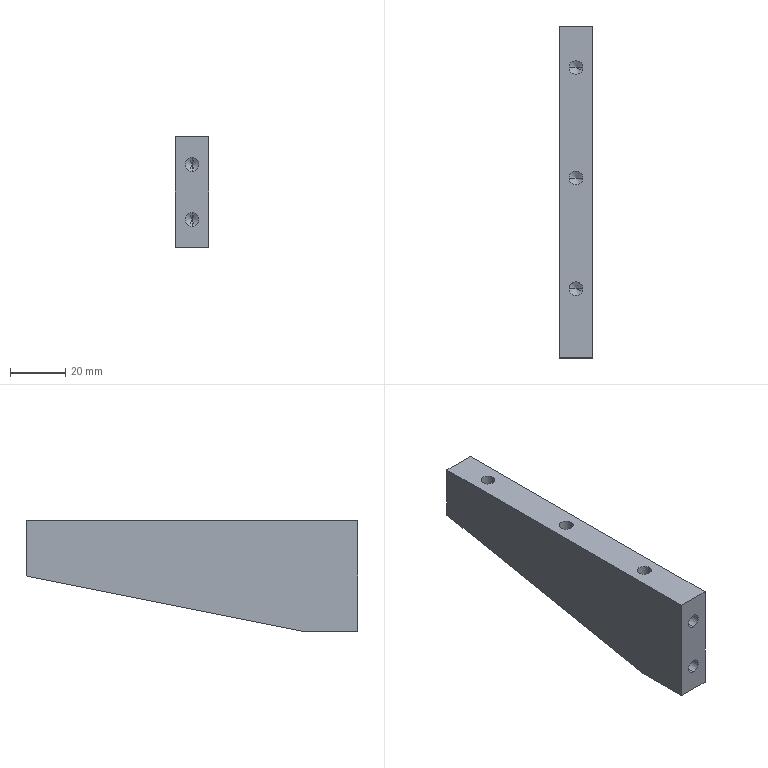Component | SolidWorks | LD101-02--Q1037-Q1-2-1 | 1 solid | 27 faces | box 12 x 120 x 40 mm | volume 43587 mm3 | cylinder 10 | cone 10 | plane 7 | commonest cylinder face diameters 5 x10 | material AL6061
build123d program:
from build123d import *

# Parameters (mm, degrees)
BOSS_EXTRUDE1_DEPTH   = 6
M6_TAPPED_HOLE1_D     = 5
M6_TAPPED_HOLE1_DEPTH = 20
M6_TAPPED_HOLE1_TIP   = 1.502
M6_TAPPED_HOLE2_D     = 5
M6_TAPPED_HOLE2_DEPTH = 20
M6_TAPPED_HOLE2_TIP   = 1.502


with BuildPart() as part:
    # Sketch1 → Boss-Extrude1 (new, symmetric)
    with BuildSketch(Plane(origin=(0, 0, 0), x_dir=(0, 0, -1), z_dir=(1, 0, 0))):
        Polygon((0, 0), (40, 0), (40, 20), (20, 120), (0, 120), align=None)
    extrude(amount=BOSS_EXTRUDE1_DEPTH, both=True)

    # M6 Tapped Hole1
    with Locations(Plane(origin=(0, 0, 0), x_dir=(-1, 0, 0), z_dir=(0, -1, 0))):
        with Locations((0, 30), (0, 10)):
            Hole(M6_TAPPED_HOLE1_D / 2, depth=M6_TAPPED_HOLE1_DEPTH)
            with Locations((0, 0, -(M6_TAPPED_HOLE1_DEPTH + M6_TAPPED_HOLE1_TIP / 2))):  # 118° drill point
                Cone(0, M6_TAPPED_HOLE1_D / 2, M6_TAPPED_HOLE1_TIP, mode=Mode.SUBTRACT)

    # M6 Tapped Hole2
    with Locations(Plane.XY):
        with Locations((0, 25), (0, 65), (0, 105)):
            Hole(M6_TAPPED_HOLE2_D / 2, depth=M6_TAPPED_HOLE2_DEPTH)
            with Locations((0, 0, -(M6_TAPPED_HOLE2_DEPTH + M6_TAPPED_HOLE2_TIP / 2))):  # 118° drill point
                Cone(0, M6_TAPPED_HOLE2_D / 2, M6_TAPPED_HOLE2_TIP, mode=Mode.SUBTRACT)


solid = part.part

# Placed as in the assembly
solid = solid.moved(Location((-494.29, -239.897, -12.743), (0, 0, 0)))
STEP:
#1=COLOUR_RGB('',0.7922,0.8196,0.9333);
#2=FILL_AREA_STYLE_COLOUR('',#1);
#3=FILL_AREA_STYLE('',(#2));
#4=SURFACE_STYLE_FILL_AREA(#3);
#5=SURFACE_SIDE_STYLE('',(#4));
#6=SURFACE_STYLE_USAGE(.BOTH.,#5);
#7=PRESENTATION_STYLE_ASSIGNMENT((#6));
#8=CARTESIAN_POINT('',(-19.559,-8.461,-1.289));
#9=VERTEX_POINT('',#8);
#10=CARTESIAN_POINT('',(-19.362,-8.461,-1.289));
#11=VERTEX_POINT('',#10);
#12=CARTESIAN_POINT('',(-19.46,-8.461,-1.289));
#13=DIRECTION('',(0.,0.,1.));
#14=DIRECTION('',(1.,0.,0.));
#15=AXIS2_PLACEMENT_3D('',#12,#13,#14);
#16=CIRCLE('',#15,0.09843);
#17=EDGE_CURVE('',#9,#11,#16,.T.);
#18=ORIENTED_EDGE('',*,*,#17,.F.);
#19=CARTESIAN_POINT('',(-19.559,-8.461,-0.5017));
#20=VERTEX_POINT('',#19);
#21=CARTESIAN_POINT('',(-19.559,-8.461,-0.5017));
#22=DIRECTION('',(0.,0.,1.));
#23=VECTOR('',#22,39.37);
#24=LINE('',#21,#23);
#25=EDGE_CURVE('',#9,#20,#24,.T.);
#26=ORIENTED_EDGE('',*,*,#25,.T.);
#27=CARTESIAN_POINT('',(-19.362,-8.461,-0.5017));
#28=VERTEX_POINT('',#27);
#29=CARTESIAN_POINT('',(-19.46,-8.461,-0.5017));
#30=DIRECTION('',(0.,0.,1.));
#31=DIRECTION('',(1.,0.,0.));
#32=AXIS2_PLACEMENT_3D('',#29,#30,#31);
#33=CIRCLE('',#32,0.09843);
#34=EDGE_CURVE('',#20,#28,#33,.T.);
#35=ORIENTED_EDGE('',*,*,#34,.T.);
#36=CARTESIAN_POINT('',(-19.362,-8.461,-0.5017));
#37=DIRECTION('',(0.,0.,1.));
#38=VECTOR('',#37,39.37);
#39=LINE('',#36,#38);
#40=EDGE_CURVE('',#11,#28,#39,.T.);
#41=ORIENTED_EDGE('',*,*,#40,.F.);
#42=EDGE_LOOP('',(#18,#26,#35,#41));
#43=FACE_OUTER_BOUND('',#42,.T.);
#44=CARTESIAN_POINT('',(-19.46,-8.461,-0.5017));
#45=DIRECTION('',(0.,0.,1.));
#46=DIRECTION('',(1.,0.,0.));
#47=AXIS2_PLACEMENT_3D('',#44,#45,#46);
#48=CYLINDRICAL_SURFACE('',#47,0.09843);
#49=ADVANCED_FACE('',(#43),#48,.F.);
#50=CARTESIAN_POINT('',(-19.46,-8.461,-1.348));
#51=VERTEX_POINT('',#50);
#52=CARTESIAN_POINT('',(-19.362,-8.461,-1.289));
#53=DIRECTION('',(0.8572,0.,0.515));
#54=VECTOR('',#53,39.37);
#55=LINE('',#52,#54);
#56=EDGE_CURVE('',#51,#11,#55,.T.);
#57=ORIENTED_EDGE('',*,*,#56,.F.);
#58=CARTESIAN_POINT('',(-19.559,-8.461,-1.289));
#59=DIRECTION('',(-0.8572,0.,0.515));
#60=VECTOR('',#59,39.37);
#61=LINE('',#58,#60);
#62=EDGE_CURVE('',#51,#9,#61,.T.);
#63=ORIENTED_EDGE('',*,*,#62,.T.);
#64=ORIENTED_EDGE('',*,*,#17,.T.);
#65=EDGE_LOOP('',(#57,#63,#64));
#66=FACE_OUTER_BOUND('',#65,.T.);
#67=CARTESIAN_POINT('',(-19.46,-8.461,-1.289));
#68=DIRECTION('',(0.,0.,1.));
#69=DIRECTION('',(1.,0.,0.));
#70=AXIS2_PLACEMENT_3D('',#67,#68,#69);
#71=CONICAL_SURFACE('',#70,0.09843,1.03);
#72=ADVANCED_FACE('',(#66),#71,.F.);
#73=CARTESIAN_POINT('',(-19.559,-6.886,-1.289));
#74=VERTEX_POINT('',#73);
#75=CARTESIAN_POINT('',(-19.362,-6.886,-1.289));
#76=VERTEX_POINT('',#75);
#77=CARTESIAN_POINT('',(-19.46,-6.886,-1.289));
#78=DIRECTION('',(0.,0.,1.));
#79=DIRECTION('',(1.,0.,0.));
#80=AXIS2_PLACEMENT_3D('',#77,#78,#79);
#81=CIRCLE('',#80,0.09843);
#82=EDGE_CURVE('',#74,#76,#81,.T.);
#83=ORIENTED_EDGE('',*,*,#82,.F.);
#84=CARTESIAN_POINT('',(-19.559,-6.886,-0.5017));
#85=VERTEX_POINT('',#84);
#86=CARTESIAN_POINT('',(-19.559,-6.886,-0.5017));
#87=DIRECTION('',(0.,0.,1.));
#88=VECTOR('',#87,39.37);
#89=LINE('',#86,#88);
#90=EDGE_CURVE('',#74,#85,#89,.T.);
#91=ORIENTED_EDGE('',*,*,#90,.T.);
#92=CARTESIAN_POINT('',(-19.362,-6.886,-0.5017));
#93=VERTEX_POINT('',#92);
#94=CARTESIAN_POINT('',(-19.46,-6.886,-0.5017));
#95=DIRECTION('',(0.,0.,1.));
#96=DIRECTION('',(1.,0.,0.));
#97=AXIS2_PLACEMENT_3D('',#94,#95,#96);
#98=CIRCLE('',#97,0.09843);
#99=EDGE_CURVE('',#85,#93,#98,.T.);
#100=ORIENTED_EDGE('',*,*,#99,.T.);
#101=CARTESIAN_POINT('',(-19.362,-6.886,-0.5017));
#102=DIRECTION('',(0.,0.,1.));
#103=VECTOR('',#102,39.37);
#104=LINE('',#101,#103);
#105=EDGE_CURVE('',#76,#93,#104,.T.);
#106=ORIENTED_EDGE('',*,*,#105,.F.);
#107=EDGE_LOOP('',(#83,#91,#100,#106));
#108=FACE_OUTER_BOUND('',#107,.T.);
#109=CARTESIAN_POINT('',(-19.46,-6.886,-0.5017));
#110=DIRECTION('',(0.,0.,1.));
#111=DIRECTION('',(1.,0.,0.));
#112=AXIS2_PLACEMENT_3D('',#109,#110,#111);
#113=CYLINDRICAL_SURFACE('',#112,0.09843);
#114=ADVANCED_FACE('',(#108),#113,.F.);
#115=CARTESIAN_POINT('',(-19.46,-6.886,-1.348));
#116=VERTEX_POINT('',#115);
#117=CARTESIAN_POINT('',(-19.362,-6.886,-1.289));
#118=DIRECTION('',(0.8572,0.,0.515));
#119=VECTOR('',#118,39.37);
#120=LINE('',#117,#119);
#121=EDGE_CURVE('',#116,#76,#120,.T.);
#122=ORIENTED_EDGE('',*,*,#121,.F.);
#123=CARTESIAN_POINT('',(-19.559,-6.886,-1.289));
#124=DIRECTION('',(-0.8572,0.,0.515));
#125=VECTOR('',#124,39.37);
#126=LINE('',#123,#125);
#127=EDGE_CURVE('',#116,#74,#126,.T.);
#128=ORIENTED_EDGE('',*,*,#127,.T.);
#129=ORIENTED_EDGE('',*,*,#82,.T.);
#130=EDGE_LOOP('',(#122,#128,#129));
#131=FACE_OUTER_BOUND('',#130,.T.);
#132=CARTESIAN_POINT('',(-19.46,-6.886,-1.289));
#133=DIRECTION('',(0.,0.,1.));
#134=DIRECTION('',(1.,0.,0.));
#135=AXIS2_PLACEMENT_3D('',#132,#133,#134);
#136=CONICAL_SURFACE('',#135,0.09843,1.03);
#137=ADVANCED_FACE('',(#131),#136,.F.);
#138=CARTESIAN_POINT('',(-19.559,-5.311,-1.289));
#139=VERTEX_POINT('',#138);
#140=CARTESIAN_POINT('',(-19.362,-5.311,-1.289));
#141=VERTEX_POINT('',#140);
#142=CARTESIAN_POINT('',(-19.46,-5.311,-1.289));
#143=DIRECTION('',(0.,0.,1.));
#144=DIRECTION('',(1.,0.,0.));
#145=AXIS2_PLACEMENT_3D('',#142,#143,#144);
#146=CIRCLE('',#145,0.09843);
#147=EDGE_CURVE('',#139,#141,#146,.T.);
#148=ORIENTED_EDGE('',*,*,#147,.F.);
#149=CARTESIAN_POINT('',(-19.559,-5.311,-0.5017));
#150=VERTEX_POINT('',#149);
#151=CARTESIAN_POINT('',(-19.559,-5.311,-0.5017));
#152=DIRECTION('',(0.,0.,1.));
#153=VECTOR('',#152,39.37);
#154=LINE('',#151,#153);
#155=EDGE_CURVE('',#139,#150,#154,.T.);
#156=ORIENTED_EDGE('',*,*,#155,.T.);
#157=CARTESIAN_POINT('',(-19.362,-5.311,-0.5017));
#158=VERTEX_POINT('',#157);
#159=CARTESIAN_POINT('',(-19.46,-5.311,-0.5017));
#160=DIRECTION('',(0.,0.,1.));
#161=DIRECTION('',(1.,0.,0.));
#162=AXIS2_PLACEMENT_3D('',#159,#160,#161);
#163=CIRCLE('',#162,0.09843);
#164=EDGE_CURVE('',#150,#158,#163,.T.);
#165=ORIENTED_EDGE('',*,*,#164,.T.);
#166=CARTESIAN_POINT('',(-19.362,-5.311,-0.5017));
#167=DIRECTION('',(0.,0.,1.));
#168=VECTOR('',#167,39.37);
#169=LINE('',#166,#168);
#170=EDGE_CURVE('',#141,#158,#169,.T.);
#171=ORIENTED_EDGE('',*,*,#170,.F.);
#172=EDGE_LOOP('',(#148,#156,#165,#171));
#173=FACE_OUTER_BOUND('',#172,.T.);
#174=CARTESIAN_POINT('',(-19.46,-5.311,-0.5017));
#175=DIRECTION('',(0.,0.,1.));
#176=DIRECTION('',(1.,0.,0.));
#177=AXIS2_PLACEMENT_3D('',#174,#175,#176);
#178=CYLINDRICAL_SURFACE('',#177,0.09843);
#179=ADVANCED_FACE('',(#173),#178,.F.);
#180=CARTESIAN_POINT('',(-19.46,-5.311,-1.348));
#181=VERTEX_POINT('',#180);
#182=CARTESIAN_POINT('',(-19.362,-5.311,-1.289));
#183=DIRECTION('',(0.8572,0.,0.515));
#184=VECTOR('',#183,39.37);
#185=LINE('',#182,#184);
#186=EDGE_CURVE('',#181,#141,#185,.T.);
#187=ORIENTED_EDGE('',*,*,#186,.F.);
#188=CARTESIAN_POINT('',(-19.559,-5.311,-1.289));
#189=DIRECTION('',(-0.8572,0.,0.515));
#190=VECTOR('',#189,39.37);
#191=LINE('',#188,#190);
#192=EDGE_CURVE('',#181,#139,#191,.T.);
#193=ORIENTED_EDGE('',*,*,#192,.T.);
#194=ORIENTED_EDGE('',*,*,#147,.T.);
#195=EDGE_LOOP('',(#187,#193,#194));
#196=FACE_OUTER_BOUND('',#195,.T.);
#197=CARTESIAN_POINT('',(-19.46,-5.311,-1.289));
#198=DIRECTION('',(0.,0.,1.));
#199=DIRECTION('',(1.,0.,0.));
#200=AXIS2_PLACEMENT_3D('',#197,#198,#199);
#201=CONICAL_SURFACE('',#200,0.09843,1.03);
#202=ADVANCED_FACE('',(#196),#201,.F.);
#203=CARTESIAN_POINT('',(-19.46,-8.657,-1.584));
#204=VERTEX_POINT('',#203);
#205=CARTESIAN_POINT('',(-19.46,-8.657,-1.781));
#206=VERTEX_POINT('',#205);
#207=CARTESIAN_POINT('',(-19.46,-8.657,-1.683));
#208=DIRECTION('',(0.,-1.,0.));
#209=DIRECTION('',(0.,0.,-1.));
#210=AXIS2_PLACEMENT_3D('',#207,#208,#209);
#211=CIRCLE('',#210,0.09843);
#212=EDGE_CURVE('',#204,#206,#211,.T.);
#213=ORIENTED_EDGE('',*,*,#212,.F.);
#214=CARTESIAN_POINT('',(-19.46,-9.445,-1.584));
#215=VERTEX_POINT('',#214);
#216=CARTESIAN_POINT('',(-19.46,-9.445,-1.584));
#217=DIRECTION('',(0.,-1.,0.));
#218=VECTOR('',#217,39.37);
#219=LINE('',#216,#218);
#220=EDGE_CURVE('',#204,#215,#219,.T.);
#221=ORIENTED_EDGE('',*,*,#220,.T.);
#222=CARTESIAN_POINT('',(-19.46,-9.445,-1.781));
#223=VERTEX_POINT('',#222);
#224=CARTESIAN_POINT('',(-19.46,-9.445,-1.683));
#225=DIRECTION('',(0.,-1.,0.));
#226=DIRECTION('',(0.,0.,-1.));
#227=AXIS2_PLACEMENT_3D('',#224,#225,#226);
#228=CIRCLE('',#227,0.09843);
#229=EDGE_CURVE('',#215,#223,#228,.T.);
#230=ORIENTED_EDGE('',*,*,#229,.T.);
#231=CARTESIAN_POINT('',(-19.46,-9.445,-1.781));
#232=DIRECTION('',(0.,-1.,0.));
#233=VECTOR('',#232,39.37);
#234=LINE('',#231,#233);
#235=EDGE_CURVE('',#206,#223,#234,.T.);
#236=ORIENTED_EDGE('',*,*,#235,.F.);
#237=EDGE_LOOP('',(#213,#221,#230,#236));
#238=FACE_OUTER_BOUND('',#237,.T.);
#239=CARTESIAN_POINT('',(-19.46,-9.445,-1.683));
#240=DIRECTION('',(0.,-1.,0.));
#241=DIRECTION('',(0.,0.,-1.));
#242=AXIS2_PLACEMENT_3D('',#239,#240,#241);
#243=CYLINDRICAL_SURFACE('',#242,0.09843);
#244=ADVANCED_FACE('',(#238),#243,.F.);
#245=CARTESIAN_POINT('',(-19.46,-8.598,-1.683));
#246=VERTEX_POINT('',#245);
#247=CARTESIAN_POINT('',(-19.46,-8.657,-1.781));
#248=DIRECTION('',(0.,-0.515,-0.8572));
#249=VECTOR('',#248,39.37);
#250=LINE('',#247,#249);
#251=EDGE_CURVE('',#246,#206,#250,.T.);
#252=ORIENTED_EDGE('',*,*,#251,.F.);
#253=CARTESIAN_POINT('',(-19.46,-8.657,-1.584));
#254=DIRECTION('',(0.,-0.515,0.8572));
#255=VECTOR('',#254,39.37);
#256=LINE('',#253,#255);
#257=EDGE_CURVE('',#246,#204,#256,.T.);
#258=ORIENTED_EDGE('',*,*,#257,.T.);
#259=ORIENTED_EDGE('',*,*,#212,.T.);
#260=EDGE_LOOP('',(#252,#258,#259));
#261=FACE_OUTER_BOUND('',#260,.T.);
#262=CARTESIAN_POINT('',(-19.46,-8.657,-1.683));
#263=DIRECTION('',(0.,-1.,0.));
#264=DIRECTION('',(0.,0.,-1.));
#265=AXIS2_PLACEMENT_3D('',#262,#263,#264);
#266=CONICAL_SURFACE('',#265,0.09843,1.03);
#267=ADVANCED_FACE('',(#261),#266,.F.);
#268=CARTESIAN_POINT('',(-19.46,-8.657,-0.797));
#269=VERTEX_POINT('',#268);
#270=CARTESIAN_POINT('',(-19.46,-8.657,-0.9938));
#271=VERTEX_POINT('',#270);
#272=CARTESIAN_POINT('',(-19.46,-8.657,-0.8954));
#273=DIRECTION('',(0.,-1.,0.));
#274=DIRECTION('',(0.,0.,-1.));
#275=AXIS2_PLACEMENT_3D('',#272,#273,#274);
#276=CIRCLE('',#275,0.09843);
#277=EDGE_CURVE('',#269,#271,#276,.T.);
#278=ORIENTED_EDGE('',*,*,#277,.F.);
#279=CARTESIAN_POINT('',(-19.46,-9.445,-0.797));
#280=VERTEX_POINT('',#279);
#281=CARTESIAN_POINT('',(-19.46,-9.445,-0.797));
#282=DIRECTION('',(0.,-1.,0.));
#283=VECTOR('',#282,39.37);
#284=LINE('',#281,#283);
#285=EDGE_CURVE('',#269,#280,#284,.T.);
#286=ORIENTED_EDGE('',*,*,#285,.T.);
#287=CARTESIAN_POINT('',(-19.46,-9.445,-0.9938));
#288=VERTEX_POINT('',#287);
#289=CARTESIAN_POINT('',(-19.46,-9.445,-0.8954));
#290=DIRECTION('',(0.,-1.,0.));
#291=DIRECTION('',(0.,0.,-1.));
#292=AXIS2_PLACEMENT_3D('',#289,#290,#291);
#293=CIRCLE('',#292,0.09843);
#294=EDGE_CURVE('',#280,#288,#293,.T.);
#295=ORIENTED_EDGE('',*,*,#294,.T.);
#296=CARTESIAN_POINT('',(-19.46,-9.445,-0.9938));
#297=DIRECTION('',(0.,-1.,0.));
#298=VECTOR('',#297,39.37);
#299=LINE('',#296,#298);
#300=EDGE_CURVE('',#271,#288,#299,.T.);
#301=ORIENTED_EDGE('',*,*,#300,.F.);
#302=EDGE_LOOP('',(#278,#286,#295,#301));
#303=FACE_OUTER_BOUND('',#302,.T.);
#304=CARTESIAN_POINT('',(-19.46,-9.445,-0.8954));
#305=DIRECTION('',(0.,-1.,0.));
#306=DIRECTION('',(0.,0.,-1.));
#307=AXIS2_PLACEMENT_3D('',#304,#305,#306);
#308=CYLINDRICAL_SURFACE('',#307,0.09843);
#309=ADVANCED_FACE('',(#303),#308,.F.);
#310=CARTESIAN_POINT('',(-19.46,-8.598,-0.8954));
#311=VERTEX_POINT('',#310);
#312=CARTESIAN_POINT('',(-19.46,-8.657,-0.9938));
#313=DIRECTION('',(0.,-0.515,-0.8572));
#314=VECTOR('',#313,39.37);
#315=LINE('',#312,#314);
#316=EDGE_CURVE('',#311,#271,#315,.T.);
#317=ORIENTED_EDGE('',*,*,#316,.F.);
#318=CARTESIAN_POINT('',(-19.46,-8.657,-0.797));
#319=DIRECTION('',(0.,-0.515,0.8572));
#320=VECTOR('',#319,39.37);
#321=LINE('',#318,#320);
#322=EDGE_CURVE('',#311,#269,#321,.T.);
#323=ORIENTED_EDGE('',*,*,#322,.T.);
#324=ORIENTED_EDGE('',*,*,#277,.T.);
#325=EDGE_LOOP('',(#317,#323,#324));
#326=FACE_OUTER_BOUND('',#325,.T.);
#327=CARTESIAN_POINT('',(-19.46,-8.657,-0.8954));
#328=DIRECTION('',(0.,-1.,0.));
#329=DIRECTION('',(0.,0.,-1.));
#330=AXIS2_PLACEMENT_3D('',#327,#328,#329);
#331=CONICAL_SURFACE('',#330,0.09843,1.03);
#332=ADVANCED_FACE('',(#326),#331,.F.);
#333=CARTESIAN_POINT('',(-19.46,-8.461,-0.5017));
#334=DIRECTION('',(0.,0.,1.));
#335=DIRECTION('',(1.,0.,0.));
#336=AXIS2_PLACEMENT_3D('',#333,#334,#335);
#337=CIRCLE('',#336,0.09843);
#338=EDGE_CURVE('',#28,#20,#337,.T.);
#339=ORIENTED_EDGE('',*,*,#338,.F.);
#340=ORIENTED_EDGE('',*,*,#34,.F.);
#341=EDGE_LOOP('',(#339,#340));
#342=FACE_BOUND('',#341,.T.);
#343=CARTESIAN_POINT('',(-19.46,-6.886,-0.5017));
#344=DIRECTION('',(0.,0.,1.));
#345=DIRECTION('',(1.,0.,0.));
#346=AXIS2_PLACEMENT_3D('',#343,#344,#345);
#347=CIRCLE('',#346,0.09843);
#348=EDGE_CURVE('',#93,#85,#347,.T.);
#349=ORIENTED_EDGE('',*,*,#348,.F.);
#350=ORIENTED_EDGE('',*,*,#99,.F.);
#351=EDGE_LOOP('',(#349,#350));
#352=FACE_BOUND('',#351,.T.);
#353=CARTESIAN_POINT('',(-19.46,-5.311,-0.5017));
#354=DIRECTION('',(0.,0.,1.));
#355=DIRECTION('',(1.,0.,0.));
#356=AXIS2_PLACEMENT_3D('',#353,#354,#355);
#357=CIRCLE('',#356,0.09843);
#358=EDGE_CURVE('',#158,#150,#357,.T.);
#359=ORIENTED_EDGE('',*,*,#358,.F.);
#360=ORIENTED_EDGE('',*,*,#164,.F.);
#361=EDGE_LOOP('',(#359,#360));
#362=FACE_BOUND('',#361,.T.);
#363=CARTESIAN_POINT('',(-19.696,-4.72,-0.5017));
#364=VERTEX_POINT('',#363);
#365=CARTESIAN_POINT('',(-19.696,-9.445,-0.5017));
#366=VERTEX_POINT('',#365);
#367=CARTESIAN_POINT('',(-19.696,-4.72,-0.5017));
#368=DIRECTION('',(0.,-1.,0.));
#369=VECTOR('',#368,39.37);
#370=LINE('',#367,#369);
#371=EDGE_CURVE('',#364,#366,#370,.T.);
#372=ORIENTED_EDGE('',*,*,#371,.T.);
#373=CARTESIAN_POINT('',(-19.224,-9.445,-0.5017));
#374=VERTEX_POINT('',#373);
#375=CARTESIAN_POINT('',(-19.224,-9.445,-0.5017));
#376=DIRECTION('',(-1.,0.,0.));
#377=VECTOR('',#376,39.37);
#378=LINE('',#375,#377);
#379=EDGE_CURVE('',#374,#366,#378,.T.);
#380=ORIENTED_EDGE('',*,*,#379,.F.);
#381=CARTESIAN_POINT('',(-19.224,-4.72,-0.5017));
#382=VERTEX_POINT('',#381);
#383=CARTESIAN_POINT('',(-19.224,-4.72,-0.5017));
#384=DIRECTION('',(0.,-1.,0.));
#385=VECTOR('',#384,39.37);
#386=LINE('',#383,#385);
#387=EDGE_CURVE('',#382,#374,#386,.T.);
#388=ORIENTED_EDGE('',*,*,#387,.F.);
#389=CARTESIAN_POINT('',(-19.224,-4.72,-0.5017));
#390=DIRECTION('',(-1.,0.,0.));
#391=VECTOR('',#390,39.37);
#392=LINE('',#389,#391);
#393=EDGE_CURVE('',#382,#364,#392,.T.);
#394=ORIENTED_EDGE('',*,*,#393,.T.);
#395=EDGE_LOOP('',(#372,#380,#388,#394));
#396=FACE_OUTER_BOUND('',#395,.T.);
#397=CARTESIAN_POINT('',(-19.224,-4.72,-0.5017));
#398=DIRECTION('',(0.,-0.,-1.));
#399=DIRECTION('',(0.,1.,-0.));
#400=AXIS2_PLACEMENT_3D('',#397,#398,#399);
#401=PLANE('',#400);
#402=ADVANCED_FACE('',(#342,#352,#362,#396),#401,.F.);
#403=CARTESIAN_POINT('',(-19.46,-9.445,-1.683));
#404=DIRECTION('',(0.,-1.,0.));
#405=DIRECTION('',(0.,0.,-1.));
#406=AXIS2_PLACEMENT_3D('',#403,#404,#405);
#407=CIRCLE('',#406,0.09843);
#408=EDGE_CURVE('',#223,#215,#407,.T.);
#409=ORIENTED_EDGE('',*,*,#408,.F.);
#410=ORIENTED_EDGE('',*,*,#229,.F.);
#411=EDGE_LOOP('',(#409,#410));
#412=FACE_BOUND('',#411,.T.);
#413=CARTESIAN_POINT('',(-19.46,-9.445,-0.8954));
#414=DIRECTION('',(0.,-1.,0.));
#415=DIRECTION('',(0.,0.,-1.));
#416=AXIS2_PLACEMENT_3D('',#413,#414,#415);
#417=CIRCLE('',#416,0.09843);
#418=EDGE_CURVE('',#288,#280,#417,.T.);
#419=ORIENTED_EDGE('',*,*,#418,.F.);
#420=ORIENTED_EDGE('',*,*,#294,.F.);
#421=EDGE_LOOP('',(#419,#420));
#422=FACE_BOUND('',#421,.T.);
#423=CARTESIAN_POINT('',(-19.696,-9.445,-2.077));
#424=VERTEX_POINT('',#423);
#425=CARTESIAN_POINT('',(-19.696,-9.445,-0.5017));
#426=DIRECTION('',(0.,0.,-1.));
#427=VECTOR('',#426,39.37);
#428=LINE('',#425,#427);
#429=EDGE_CURVE('',#366,#424,#428,.T.);
#430=ORIENTED_EDGE('',*,*,#429,.T.);
#431=CARTESIAN_POINT('',(-19.224,-9.445,-2.077));
#432=VERTEX_POINT('',#431);
#433=CARTESIAN_POINT('',(-19.224,-9.445,-2.077));
#434=DIRECTION('',(-1.,0.,0.));
#435=VECTOR('',#434,39.37);
#436=LINE('',#433,#435);
#437=EDGE_CURVE('',#432,#424,#436,.T.);
#438=ORIENTED_EDGE('',*,*,#437,.F.);
#439=CARTESIAN_POINT('',(-19.224,-9.445,-0.5017));
#440=DIRECTION('',(0.,0.,-1.));
#441=VECTOR('',#440,39.37);
#442=LINE('',#439,#441);
#443=EDGE_CURVE('',#374,#432,#442,.T.);
#444=ORIENTED_EDGE('',*,*,#443,.F.);
#445=ORIENTED_EDGE('',*,*,#379,.T.);
#446=EDGE_LOOP('',(#430,#438,#444,#445));
#447=FACE_OUTER_BOUND('',#446,.T.);
#448=CARTESIAN_POINT('',(-19.224,-9.445,-0.5017));
#449=DIRECTION('',(0.,1.,0.));
#450=DIRECTION('',(0.,0.,1.));
#451=AXIS2_PLACEMENT_3D('',#448,#449,#450);
#452=PLANE('',#451);
#453=ADVANCED_FACE('',(#412,#422,#447),#452,.F.);
#454=CARTESIAN_POINT('',(-19.696,-8.657,-2.077));
#455=VERTEX_POINT('',#454);
#456=CARTESIAN_POINT('',(-19.696,-9.445,-2.077));
#457=DIRECTION('',(0.,1.,0.));
#458=VECTOR('',#457,39.37);
#459=LINE('',#456,#458);
#460=EDGE_CURVE('',#424,#455,#459,.T.);
#461=ORIENTED_EDGE('',*,*,#460,.T.);
#462=CARTESIAN_POINT('',(-19.224,-8.657,-2.077));
#463=VERTEX_POINT('',#462);
#464=CARTESIAN_POINT('',(-19.224,-8.657,-2.077));
#465=DIRECTION('',(-1.,0.,0.));
#466=VECTOR('',#465,39.37);
#467=LINE('',#464,#466);
#468=EDGE_CURVE('',#463,#455,#467,.T.);
#469=ORIENTED_EDGE('',*,*,#468,.F.);
#470=CARTESIAN_POINT('',(-19.224,-9.445,-2.077));
#471=DIRECTION('',(0.,1.,0.));
#472=VECTOR('',#471,39.37);
#473=LINE('',#470,#472);
#474=EDGE_CURVE('',#432,#463,#473,.T.);
#475=ORIENTED_EDGE('',*,*,#474,.F.);
#476=ORIENTED_EDGE('',*,*,#437,.T.);
#477=EDGE_LOOP('',(#461,#469,#475,#476));
#478=FACE_OUTER_BOUND('',#477,.T.);
#479=CARTESIAN_POINT('',(-19.224,-9.445,-2.077));
#480=DIRECTION('',(0.,0.,1.));
#481=DIRECTION('',(1.,0.,0.));
#482=AXIS2_PLACEMENT_3D('',#479,#480,#481);
#483=PLANE('',#482);
#484=ADVANCED_FACE('',(#478),#483,.F.);
#485=CARTESIAN_POINT('',(-19.696,-4.72,-1.289));
#486=VERTEX_POINT('',#485);
#487=CARTESIAN_POINT('',(-19.696,-8.657,-2.077));
#488=DIRECTION('',(0.,0.9806,0.1961));
#489=VECTOR('',#488,39.37);
#490=LINE('',#487,#489);
#491=EDGE_CURVE('',#455,#486,#490,.T.);
#492=ORIENTED_EDGE('',*,*,#491,.T.);
#493=CARTESIAN_POINT('',(-19.224,-4.72,-1.289));
#494=VERTEX_POINT('',#493);
#495=CARTESIAN_POINT('',(-19.224,-4.72,-1.289));
#496=DIRECTION('',(-1.,0.,0.));
#497=VECTOR('',#496,39.37);
#498=LINE('',#495,#497);
#499=EDGE_CURVE('',#494,#486,#498,.T.);
#500=ORIENTED_EDGE('',*,*,#499,.F.);
#501=CARTESIAN_POINT('',(-19.224,-8.657,-2.077));
#502=DIRECTION('',(0.,0.9806,0.1961));
#503=VECTOR('',#502,39.37);
#504=LINE('',#501,#503);
#505=EDGE_CURVE('',#463,#494,#504,.T.);
#506=ORIENTED_EDGE('',*,*,#505,.F.);
#507=ORIENTED_EDGE('',*,*,#468,.T.);
#508=EDGE_LOOP('',(#492,#500,#506,#507));
#509=FACE_OUTER_BOUND('',#508,.T.);
#510=CARTESIAN_POINT('',(-19.224,-8.657,-2.077));
#511=DIRECTION('',(0.,-0.1961,0.9806));
#512=DIRECTION('',(0.,-0.9806,-0.1961));
#513=AXIS2_PLACEMENT_3D('',#510,#511,#512);
#514=PLANE('',#513);
#515=ADVANCED_FACE('',(#509),#514,.F.);
#516=CARTESIAN_POINT('',(-19.696,-4.72,-1.289));
#517=DIRECTION('',(0.,0.,1.));
#518=VECTOR('',#517,39.37);
#519=LINE('',#516,#518);
#520=EDGE_CURVE('',#486,#364,#519,.T.);
#521=ORIENTED_EDGE('',*,*,#520,.T.);
#522=ORIENTED_EDGE('',*,*,#393,.F.);
#523=CARTESIAN_POINT('',(-19.224,-4.72,-1.289));
#524=DIRECTION('',(0.,0.,1.));
#525=VECTOR('',#524,39.37);
#526=LINE('',#523,#525);
#527=EDGE_CURVE('',#494,#382,#526,.T.);
#528=ORIENTED_EDGE('',*,*,#527,.F.);
#529=ORIENTED_EDGE('',*,*,#499,.T.);
#530=EDGE_LOOP('',(#521,#522,#528,#529));
#531=FACE_OUTER_BOUND('',#530,.T.);
#532=CARTESIAN_POINT('',(-19.224,-4.72,-1.289));
#533=DIRECTION('',(0.,-1.,0.));
#534=DIRECTION('',(0.,0.,-1.));
#535=AXIS2_PLACEMENT_3D('',#532,#533,#534);
#536=PLANE('',#535);
#537=ADVANCED_FACE('',(#531),#536,.F.);
#538=ORIENTED_EDGE('',*,*,#387,.T.);
#539=ORIENTED_EDGE('',*,*,#443,.T.);
#540=ORIENTED_EDGE('',*,*,#474,.T.);
#541=ORIENTED_EDGE('',*,*,#505,.T.);
#542=ORIENTED_EDGE('',*,*,#527,.T.);
#543=EDGE_LOOP('',(#538,#539,#540,#541,#542));
#544=FACE_OUTER_BOUND('',#543,.T.);
#545=CARTESIAN_POINT('',(-19.224,-9.445,-0.5017));
#546=DIRECTION('',(1.,0.,0.));
#547=DIRECTION('',(0.,0.,-1.));
#548=AXIS2_PLACEMENT_3D('',#545,#546,#547);
#549=PLANE('',#548);
#550=ADVANCED_FACE('',(#544),#549,.T.);
#551=ORIENTED_EDGE('',*,*,#371,.F.);
#552=ORIENTED_EDGE('',*,*,#520,.F.);
#553=ORIENTED_EDGE('',*,*,#491,.F.);
#554=ORIENTED_EDGE('',*,*,#460,.F.);
#555=ORIENTED_EDGE('',*,*,#429,.F.);
#556=EDGE_LOOP('',(#551,#552,#553,#554,#555));
#557=FACE_OUTER_BOUND('',#556,.T.);
#558=CARTESIAN_POINT('',(-19.696,-9.445,-0.5017));
#559=DIRECTION('',(1.,0.,0.));
#560=DIRECTION('',(0.,0.,-1.));
#561=AXIS2_PLACEMENT_3D('',#558,#559,#560);
#562=PLANE('',#561);
#563=ADVANCED_FACE('',(#557),#562,.F.);
#564=ORIENTED_EDGE('',*,*,#322,.F.);
#565=ORIENTED_EDGE('',*,*,#316,.T.);
#566=CARTESIAN_POINT('',(-19.46,-8.657,-0.8954));
#567=DIRECTION('',(0.,-1.,0.));
#568=DIRECTION('',(0.,0.,-1.));
#569=AXIS2_PLACEMENT_3D('',#566,#567,#568);
#570=CIRCLE('',#569,0.09843);
#571=EDGE_CURVE('',#271,#269,#570,.T.);
#572=ORIENTED_EDGE('',*,*,#571,.T.);
#573=EDGE_LOOP('',(#564,#565,#572));
#574=FACE_OUTER_BOUND('',#573,.T.);
#575=CARTESIAN_POINT('',(-19.46,-8.657,-0.8954));
#576=DIRECTION('',(0.,-1.,0.));
#577=DIRECTION('',(0.,0.,-1.));
#578=AXIS2_PLACEMENT_3D('',#575,#576,#577);
#579=CONICAL_SURFACE('',#578,0.09843,1.03);
#580=ADVANCED_FACE('',(#574),#579,.F.);
#581=ORIENTED_EDGE('',*,*,#285,.F.);
#582=ORIENTED_EDGE('',*,*,#571,.F.);
#583=ORIENTED_EDGE('',*,*,#300,.T.);
#584=ORIENTED_EDGE('',*,*,#418,.T.);
#585=EDGE_LOOP('',(#581,#582,#583,#584));
#586=FACE_OUTER_BOUND('',#585,.T.);
#587=CARTESIAN_POINT('',(-19.46,-9.445,-0.8954));
#588=DIRECTION('',(0.,-1.,0.));
#589=DIRECTION('',(0.,0.,-1.));
#590=AXIS2_PLACEMENT_3D('',#587,#588,#589);
#591=CYLINDRICAL_SURFACE('',#590,0.09843);
#592=ADVANCED_FACE('',(#586),#591,.F.);
#593=ORIENTED_EDGE('',*,*,#257,.F.);
#594=ORIENTED_EDGE('',*,*,#251,.T.);
#595=CARTESIAN_POINT('',(-19.46,-8.657,-1.683));
#596=DIRECTION('',(0.,-1.,0.));
#597=DIRECTION('',(0.,0.,-1.));
#598=AXIS2_PLACEMENT_3D('',#595,#596,#597);
#599=CIRCLE('',#598,0.09843);
#600=EDGE_CURVE('',#206,#204,#599,.T.);
#601=ORIENTED_EDGE('',*,*,#600,.T.);
#602=EDGE_LOOP('',(#593,#594,#601));
#603=FACE_OUTER_BOUND('',#602,.T.);
#604=CARTESIAN_POINT('',(-19.46,-8.657,-1.683));
#605=DIRECTION('',(0.,-1.,0.));
#606=DIRECTION('',(0.,0.,-1.));
#607=AXIS2_PLACEMENT_3D('',#604,#605,#606);
#608=CONICAL_SURFACE('',#607,0.09843,1.03);
#609=ADVANCED_FACE('',(#603),#608,.F.);
#610=ORIENTED_EDGE('',*,*,#220,.F.);
#611=ORIENTED_EDGE('',*,*,#600,.F.);
#612=ORIENTED_EDGE('',*,*,#235,.T.);
#613=ORIENTED_EDGE('',*,*,#408,.T.);
#614=EDGE_LOOP('',(#610,#611,#612,#613));
#615=FACE_OUTER_BOUND('',#614,.T.);
#616=CARTESIAN_POINT('',(-19.46,-9.445,-1.683));
#617=DIRECTION('',(0.,-1.,0.));
#618=DIRECTION('',(0.,0.,-1.));
#619=AXIS2_PLACEMENT_3D('',#616,#617,#618);
#620=CYLINDRICAL_SURFACE('',#619,0.09843);
#621=ADVANCED_FACE('',(#615),#620,.F.);
#622=ORIENTED_EDGE('',*,*,#192,.F.);
#623=ORIENTED_EDGE('',*,*,#186,.T.);
#624=CARTESIAN_POINT('',(-19.46,-5.311,-1.289));
#625=DIRECTION('',(0.,0.,1.));
#626=DIRECTION('',(1.,0.,0.));
#627=AXIS2_PLACEMENT_3D('',#624,#625,#626);
#628=CIRCLE('',#627,0.09843);
#629=EDGE_CURVE('',#141,#139,#628,.T.);
#630=ORIENTED_EDGE('',*,*,#629,.T.);
#631=EDGE_LOOP('',(#622,#623,#630));
#632=FACE_OUTER_BOUND('',#631,.T.);
#633=CARTESIAN_POINT('',(-19.46,-5.311,-1.289));
#634=DIRECTION('',(0.,0.,1.));
#635=DIRECTION('',(1.,0.,0.));
#636=AXIS2_PLACEMENT_3D('',#633,#634,#635);
#637=CONICAL_SURFACE('',#636,0.09843,1.03);
#638=ADVANCED_FACE('',(#632),#637,.F.);
#639=ORIENTED_EDGE('',*,*,#155,.F.);
#640=ORIENTED_EDGE('',*,*,#629,.F.);
#641=ORIENTED_EDGE('',*,*,#170,.T.);
#642=ORIENTED_EDGE('',*,*,#358,.T.);
#643=EDGE_LOOP('',(#639,#640,#641,#642));
#644=FACE_OUTER_BOUND('',#643,.T.);
#645=CARTESIAN_POINT('',(-19.46,-5.311,-0.5017));
#646=DIRECTION('',(0.,0.,1.));
#647=DIRECTION('',(1.,0.,0.));
#648=AXIS2_PLACEMENT_3D('',#645,#646,#647);
#649=CYLINDRICAL_SURFACE('',#648,0.09843);
#650=ADVANCED_FACE('',(#644),#649,.F.);
#651=ORIENTED_EDGE('',*,*,#127,.F.);
#652=ORIENTED_EDGE('',*,*,#121,.T.);
#653=CARTESIAN_POINT('',(-19.46,-6.886,-1.289));
#654=DIRECTION('',(0.,0.,1.));
#655=DIRECTION('',(1.,0.,0.));
#656=AXIS2_PLACEMENT_3D('',#653,#654,#655);
#657=CIRCLE('',#656,0.09843);
#658=EDGE_CURVE('',#76,#74,#657,.T.);
#659=ORIENTED_EDGE('',*,*,#658,.T.);
#660=EDGE_LOOP('',(#651,#652,#659));
#661=FACE_OUTER_BOUND('',#660,.T.);
#662=CARTESIAN_POINT('',(-19.46,-6.886,-1.289));
#663=DIRECTION('',(0.,0.,1.));
#664=DIRECTION('',(1.,0.,0.));
#665=AXIS2_PLACEMENT_3D('',#662,#663,#664);
#666=CONICAL_SURFACE('',#665,0.09843,1.03);
#667=ADVANCED_FACE('',(#661),#666,.F.);
#668=ORIENTED_EDGE('',*,*,#90,.F.);
#669=ORIENTED_EDGE('',*,*,#658,.F.);
#670=ORIENTED_EDGE('',*,*,#105,.T.);
#671=ORIENTED_EDGE('',*,*,#348,.T.);
#672=EDGE_LOOP('',(#668,#669,#670,#671));
#673=FACE_OUTER_BOUND('',#672,.T.);
#674=CARTESIAN_POINT('',(-19.46,-6.886,-0.5017));
#675=DIRECTION('',(0.,0.,1.));
#676=DIRECTION('',(1.,0.,0.));
#677=AXIS2_PLACEMENT_3D('',#674,#675,#676);
#678=CYLINDRICAL_SURFACE('',#677,0.09843);
#679=ADVANCED_FACE('',(#673),#678,.F.);
#680=ORIENTED_EDGE('',*,*,#62,.F.);
#681=ORIENTED_EDGE('',*,*,#56,.T.);
#682=CARTESIAN_POINT('',(-19.46,-8.461,-1.289));
#683=DIRECTION('',(0.,0.,1.));
#684=DIRECTION('',(1.,0.,0.));
#685=AXIS2_PLACEMENT_3D('',#682,#683,#684);
#686=CIRCLE('',#685,0.09843);
#687=EDGE_CURVE('',#11,#9,#686,.T.);
#688=ORIENTED_EDGE('',*,*,#687,.T.);
#689=EDGE_LOOP('',(#680,#681,#688));
#690=FACE_OUTER_BOUND('',#689,.T.);
#691=CARTESIAN_POINT('',(-19.46,-8.461,-1.289));
#692=DIRECTION('',(0.,0.,1.));
#693=DIRECTION('',(1.,0.,0.));
#694=AXIS2_PLACEMENT_3D('',#691,#692,#693);
#695=CONICAL_SURFACE('',#694,0.09843,1.03);
#696=ADVANCED_FACE('',(#690),#695,.F.);
#697=ORIENTED_EDGE('',*,*,#25,.F.);
#698=ORIENTED_EDGE('',*,*,#687,.F.);
#699=ORIENTED_EDGE('',*,*,#40,.T.);
#700=ORIENTED_EDGE('',*,*,#338,.T.);
#701=EDGE_LOOP('',(#697,#698,#699,#700));
#702=FACE_OUTER_BOUND('',#701,.T.);
#703=CARTESIAN_POINT('',(-19.46,-8.461,-0.5017));
#704=DIRECTION('',(0.,0.,1.));
#705=DIRECTION('',(1.,0.,0.));
#706=AXIS2_PLACEMENT_3D('',#703,#704,#705);
#707=CYLINDRICAL_SURFACE('',#706,0.09843);
#708=ADVANCED_FACE('',(#702),#707,.F.);
#709=CLOSED_SHELL('',(#49,#72,#114,#137,#179,#202,#244,#267,#309,#332,#402,#453,#484,#515,#537,#550,#563,#580,#592,#609,#621,#638,#650,#667,#679,#696,#708));
#710=MANIFOLD_SOLID_BREP('',#709);
#711=STYLED_ITEM('',(#7),#710);
#712=PRESENTATION_LAYER_ASSIGNMENT('','',(#711));
#713=CARTESIAN_POINT('',(0.,0.,0.));
#714=DIRECTION('',(0.,0.,1.));
#715=DIRECTION('',(1.,0.,0.));
#716=AXIS2_PLACEMENT_3D('',#713,#714,#715);
#717=(LENGTH_UNIT()NAMED_UNIT(*)SI_UNIT($,.METRE.));
#718=LENGTH_MEASURE_WITH_UNIT(LENGTH_MEASURE(0.0254),#717);
#719=DIMENSIONAL_EXPONENTS(1.,0.,0.,0.,0.,0.,0.);
#720=(CONVERSION_BASED_UNIT('',#718)LENGTH_UNIT()NAMED_UNIT(#719));
#721=UNCERTAINTY_MEASURE_WITH_UNIT(LENGTH_MEASURE(0.00001),#720,'','');
#722=(NAMED_UNIT(*)PLANE_ANGLE_UNIT()SI_UNIT($,.RADIAN.));
#723=(NAMED_UNIT(*)SI_UNIT($,.STERADIAN.)SOLID_ANGLE_UNIT());
#724=(GEOMETRIC_REPRESENTATION_CONTEXT(3)GLOBAL_UNCERTAINTY_ASSIGNED_CONTEXT((#721))GLOBAL_UNIT_ASSIGNED_CONTEXT((#720,#722,#723))REPRESENTATION_CONTEXT('',''));
#725=ADVANCED_BREP_SHAPE_REPRESENTATION('',(#710,#716),#724);
#726=(LENGTH_UNIT()NAMED_UNIT(*)SI_UNIT($,.METRE.));
#727=LENGTH_MEASURE_WITH_UNIT(LENGTH_MEASURE(0.0254),#726);
#728=DIMENSIONAL_EXPONENTS(1.,0.,0.,0.,0.,0.,0.);
#729=(CONVERSION_BASED_UNIT('',#727)LENGTH_UNIT()NAMED_UNIT(#728));
#730=UNCERTAINTY_MEASURE_WITH_UNIT(LENGTH_MEASURE(0.00001),#729,'','');
#731=(NAMED_UNIT(*)PLANE_ANGLE_UNIT()SI_UNIT($,.RADIAN.));
#732=(NAMED_UNIT(*)SI_UNIT($,.STERADIAN.)SOLID_ANGLE_UNIT());
#733=(GEOMETRIC_REPRESENTATION_CONTEXT(3)GLOBAL_UNCERTAINTY_ASSIGNED_CONTEXT((#730))GLOBAL_UNIT_ASSIGNED_CONTEXT((#729,#731,#732))REPRESENTATION_CONTEXT('',''));
#734=MECHANICAL_DESIGN_GEOMETRIC_PRESENTATION_REPRESENTATION('',(#711),#733);